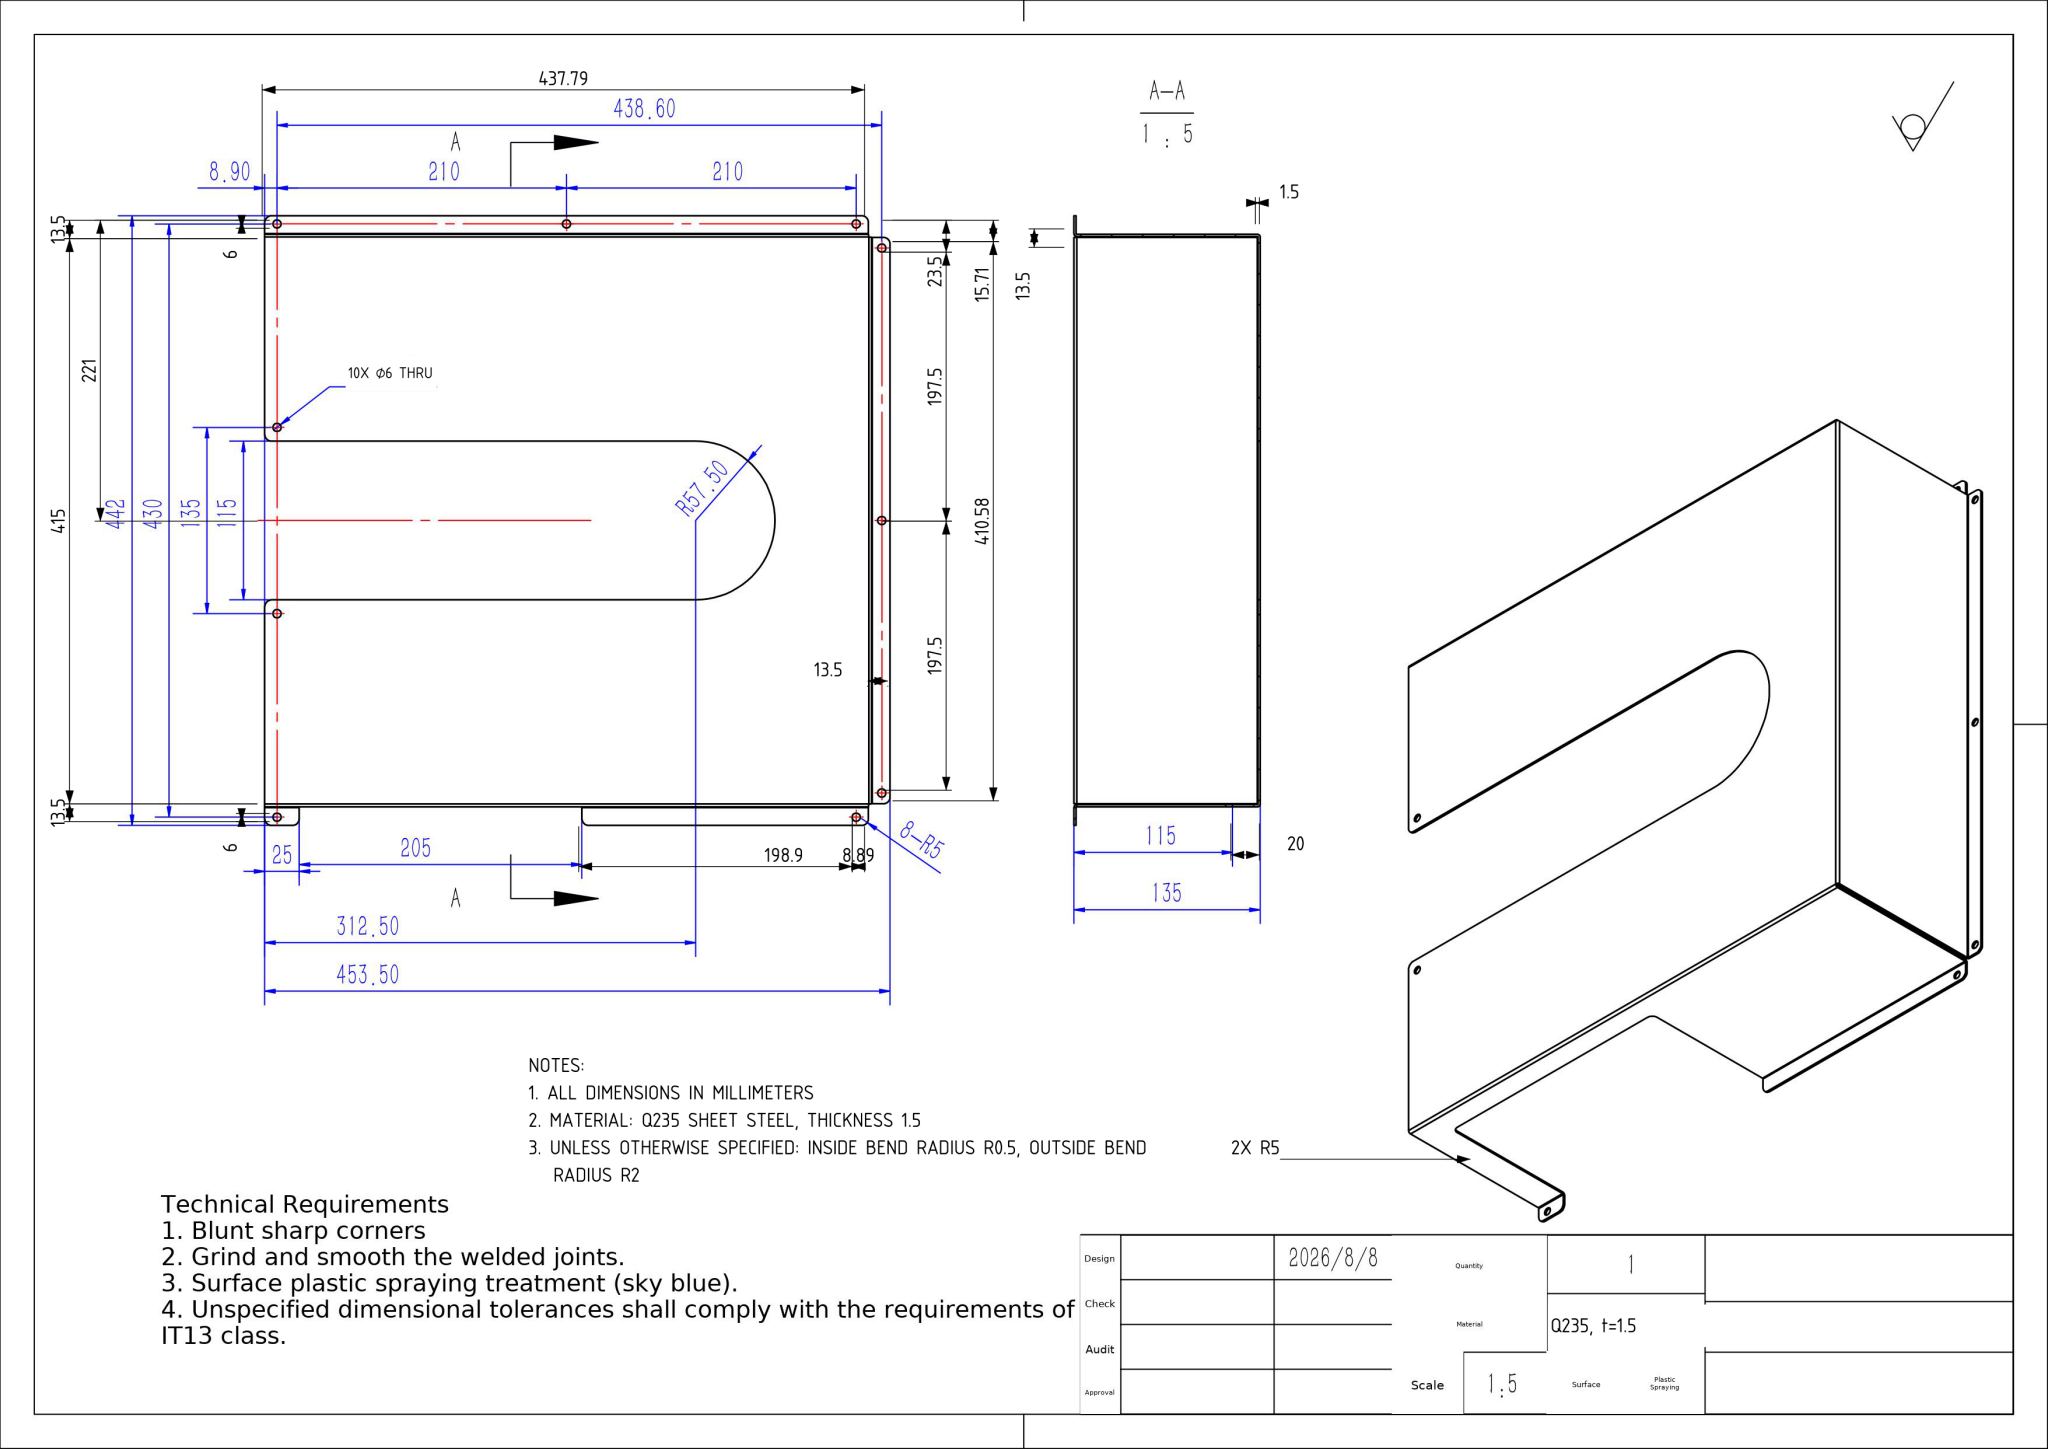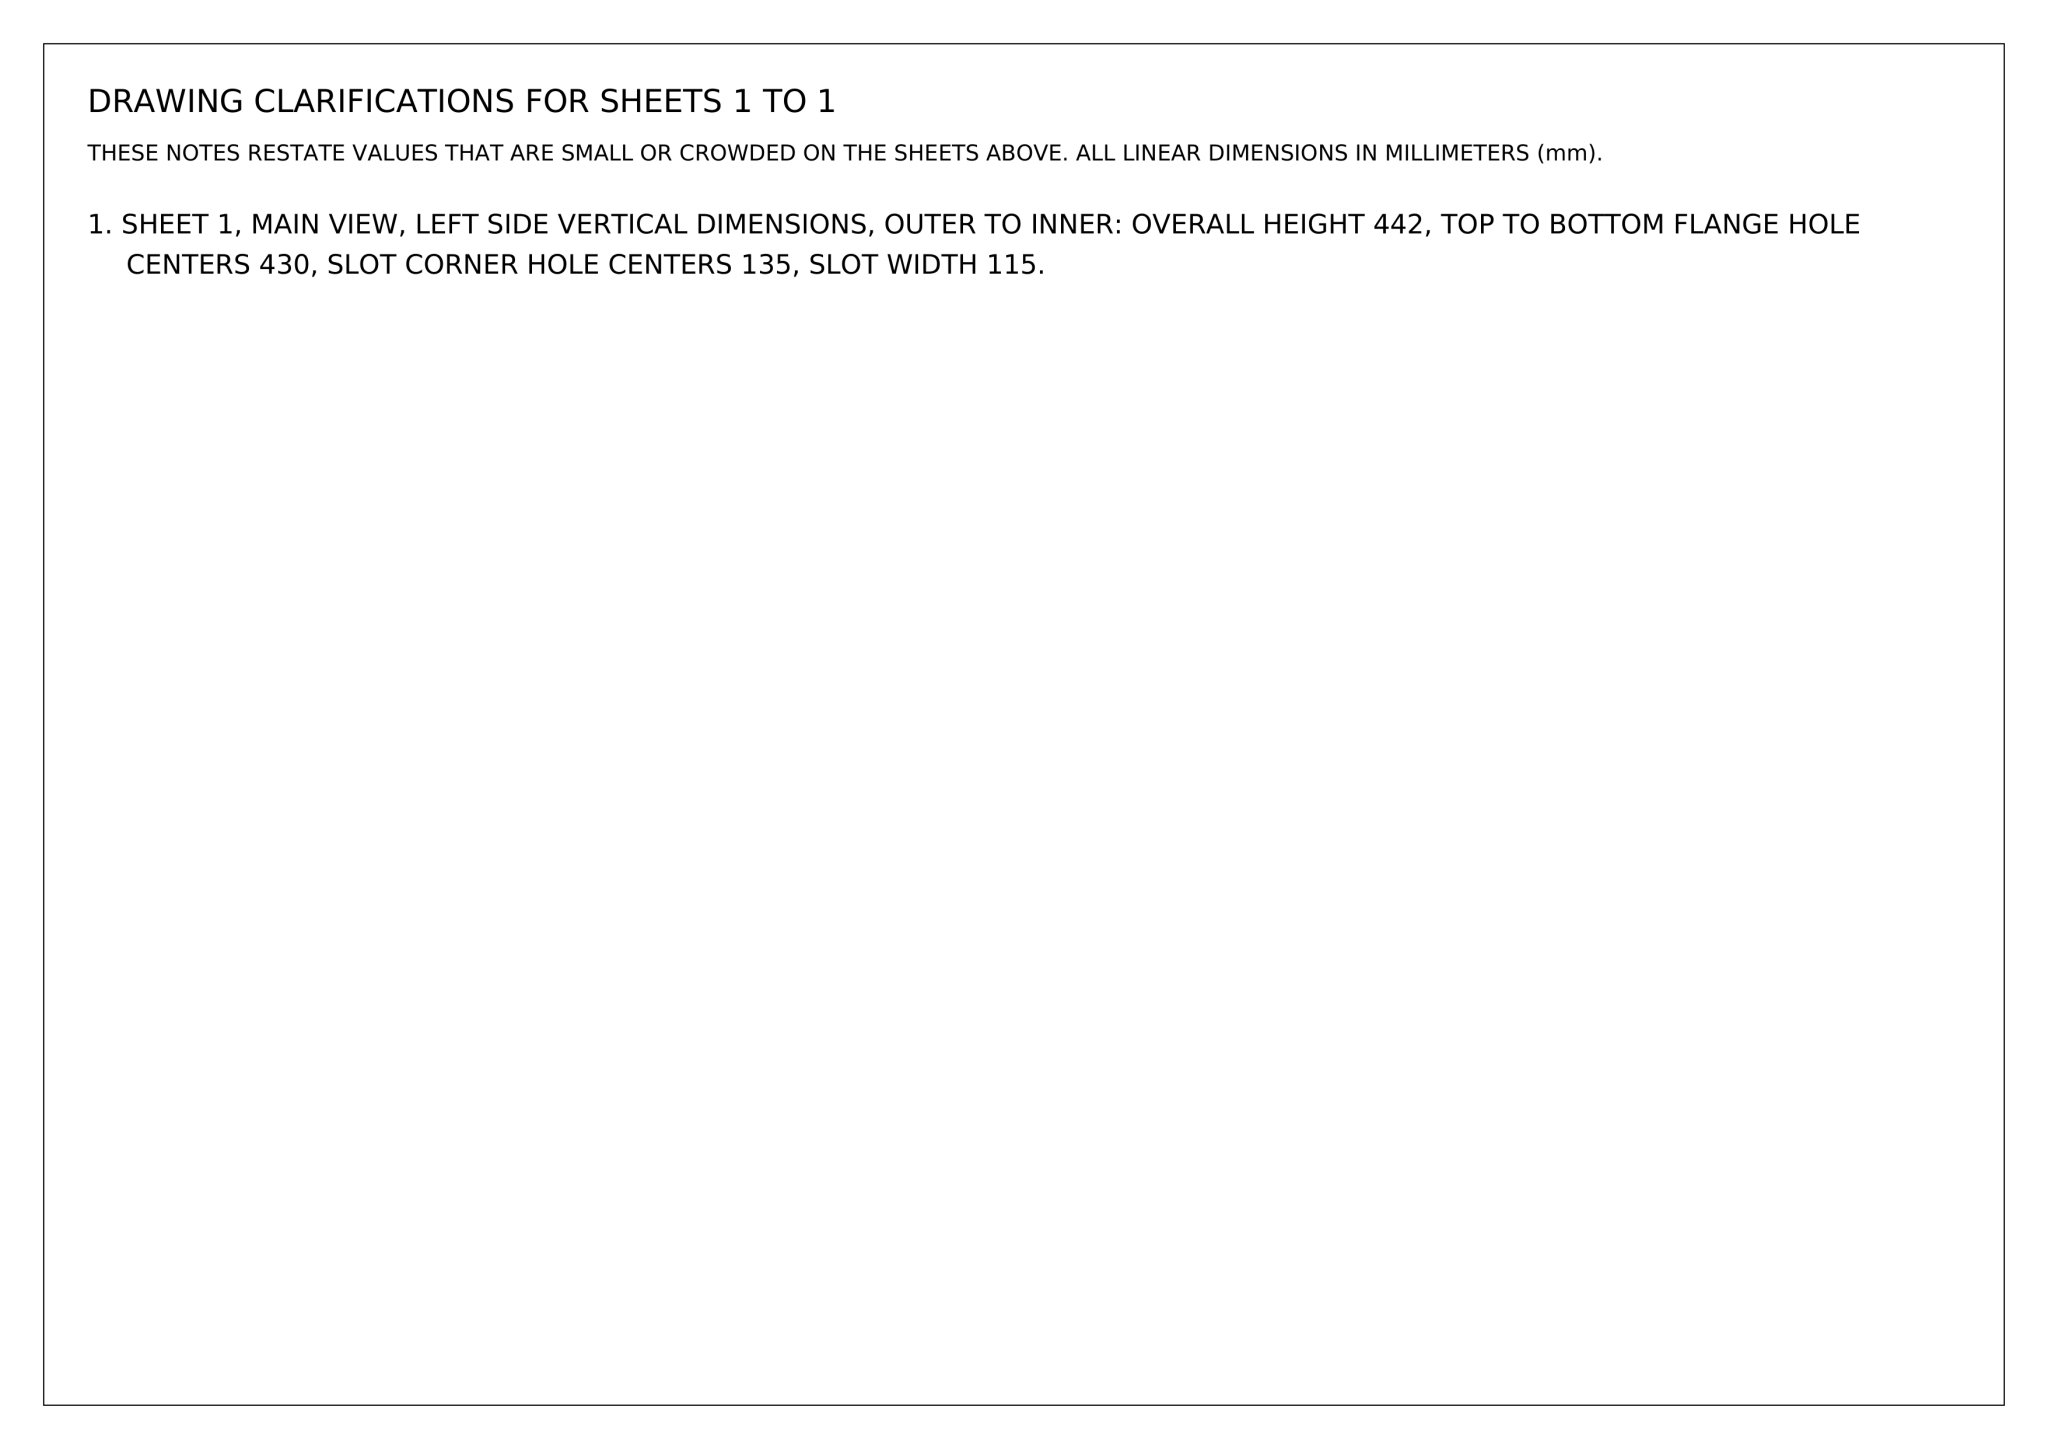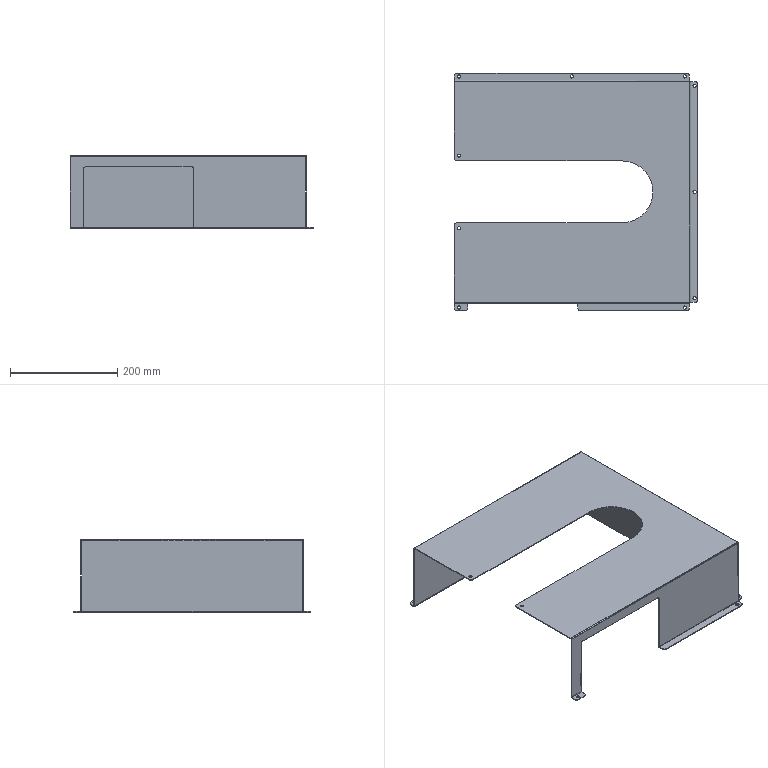Part | NX | mm | U-Notch Rectangular Equipment Enclosure | 1 solid | 103 faces | box 453.5 x 442 x 135 mm | volume 453884 mm3 | plane 51 | cylinder 48 | spline 4 | commonest cylinder face diameters 6 x20 10 x12 4 x7 1 x7 115 x2